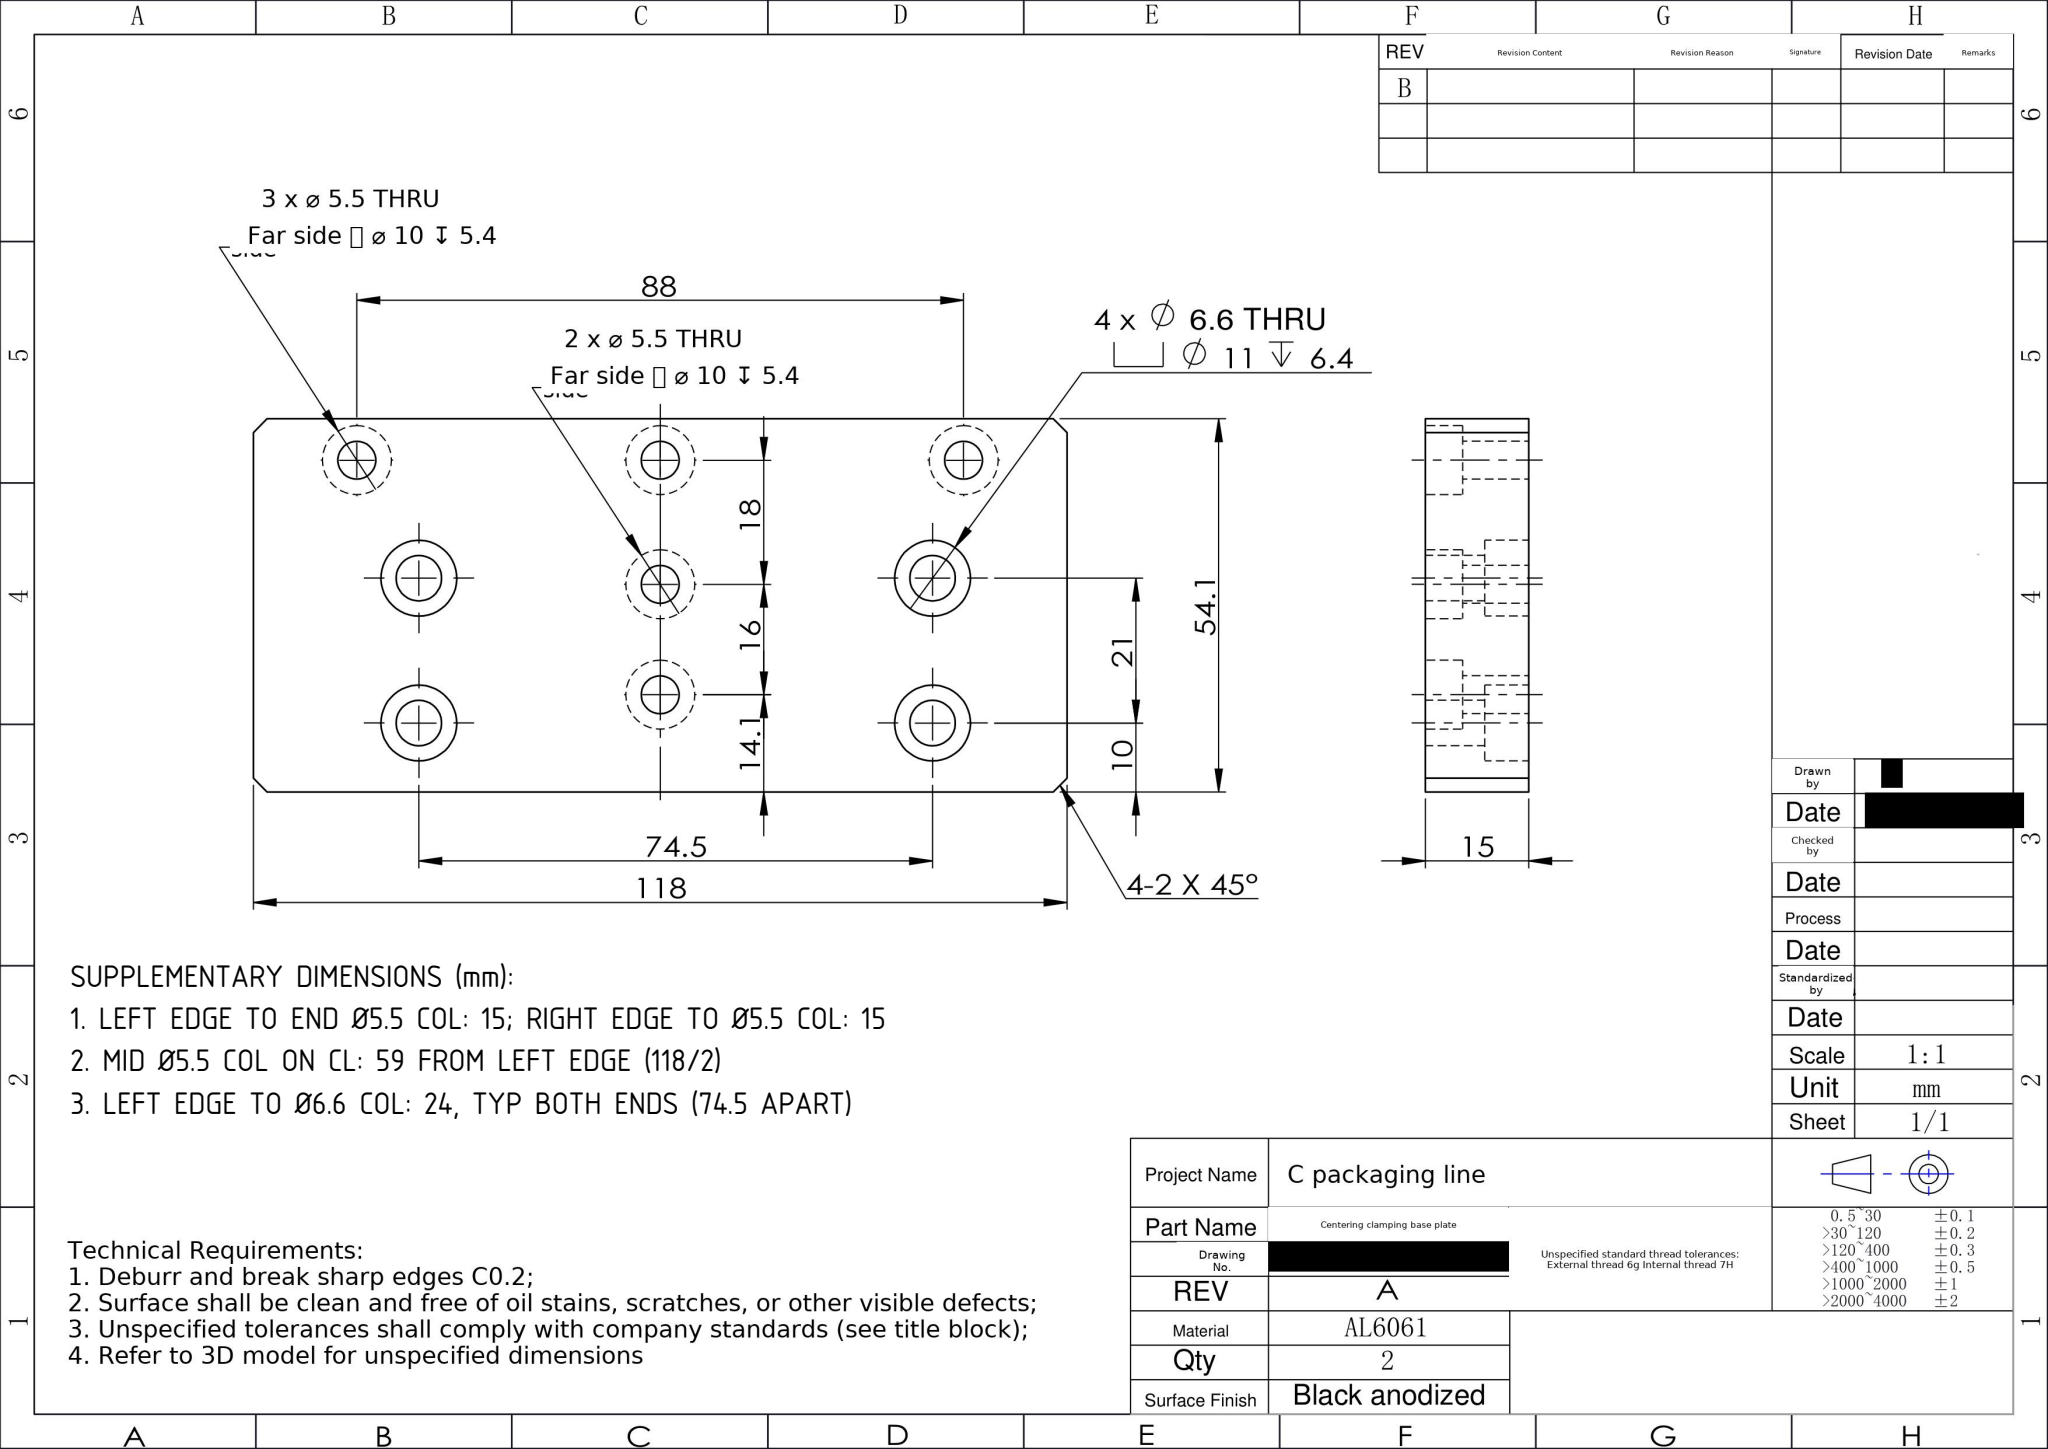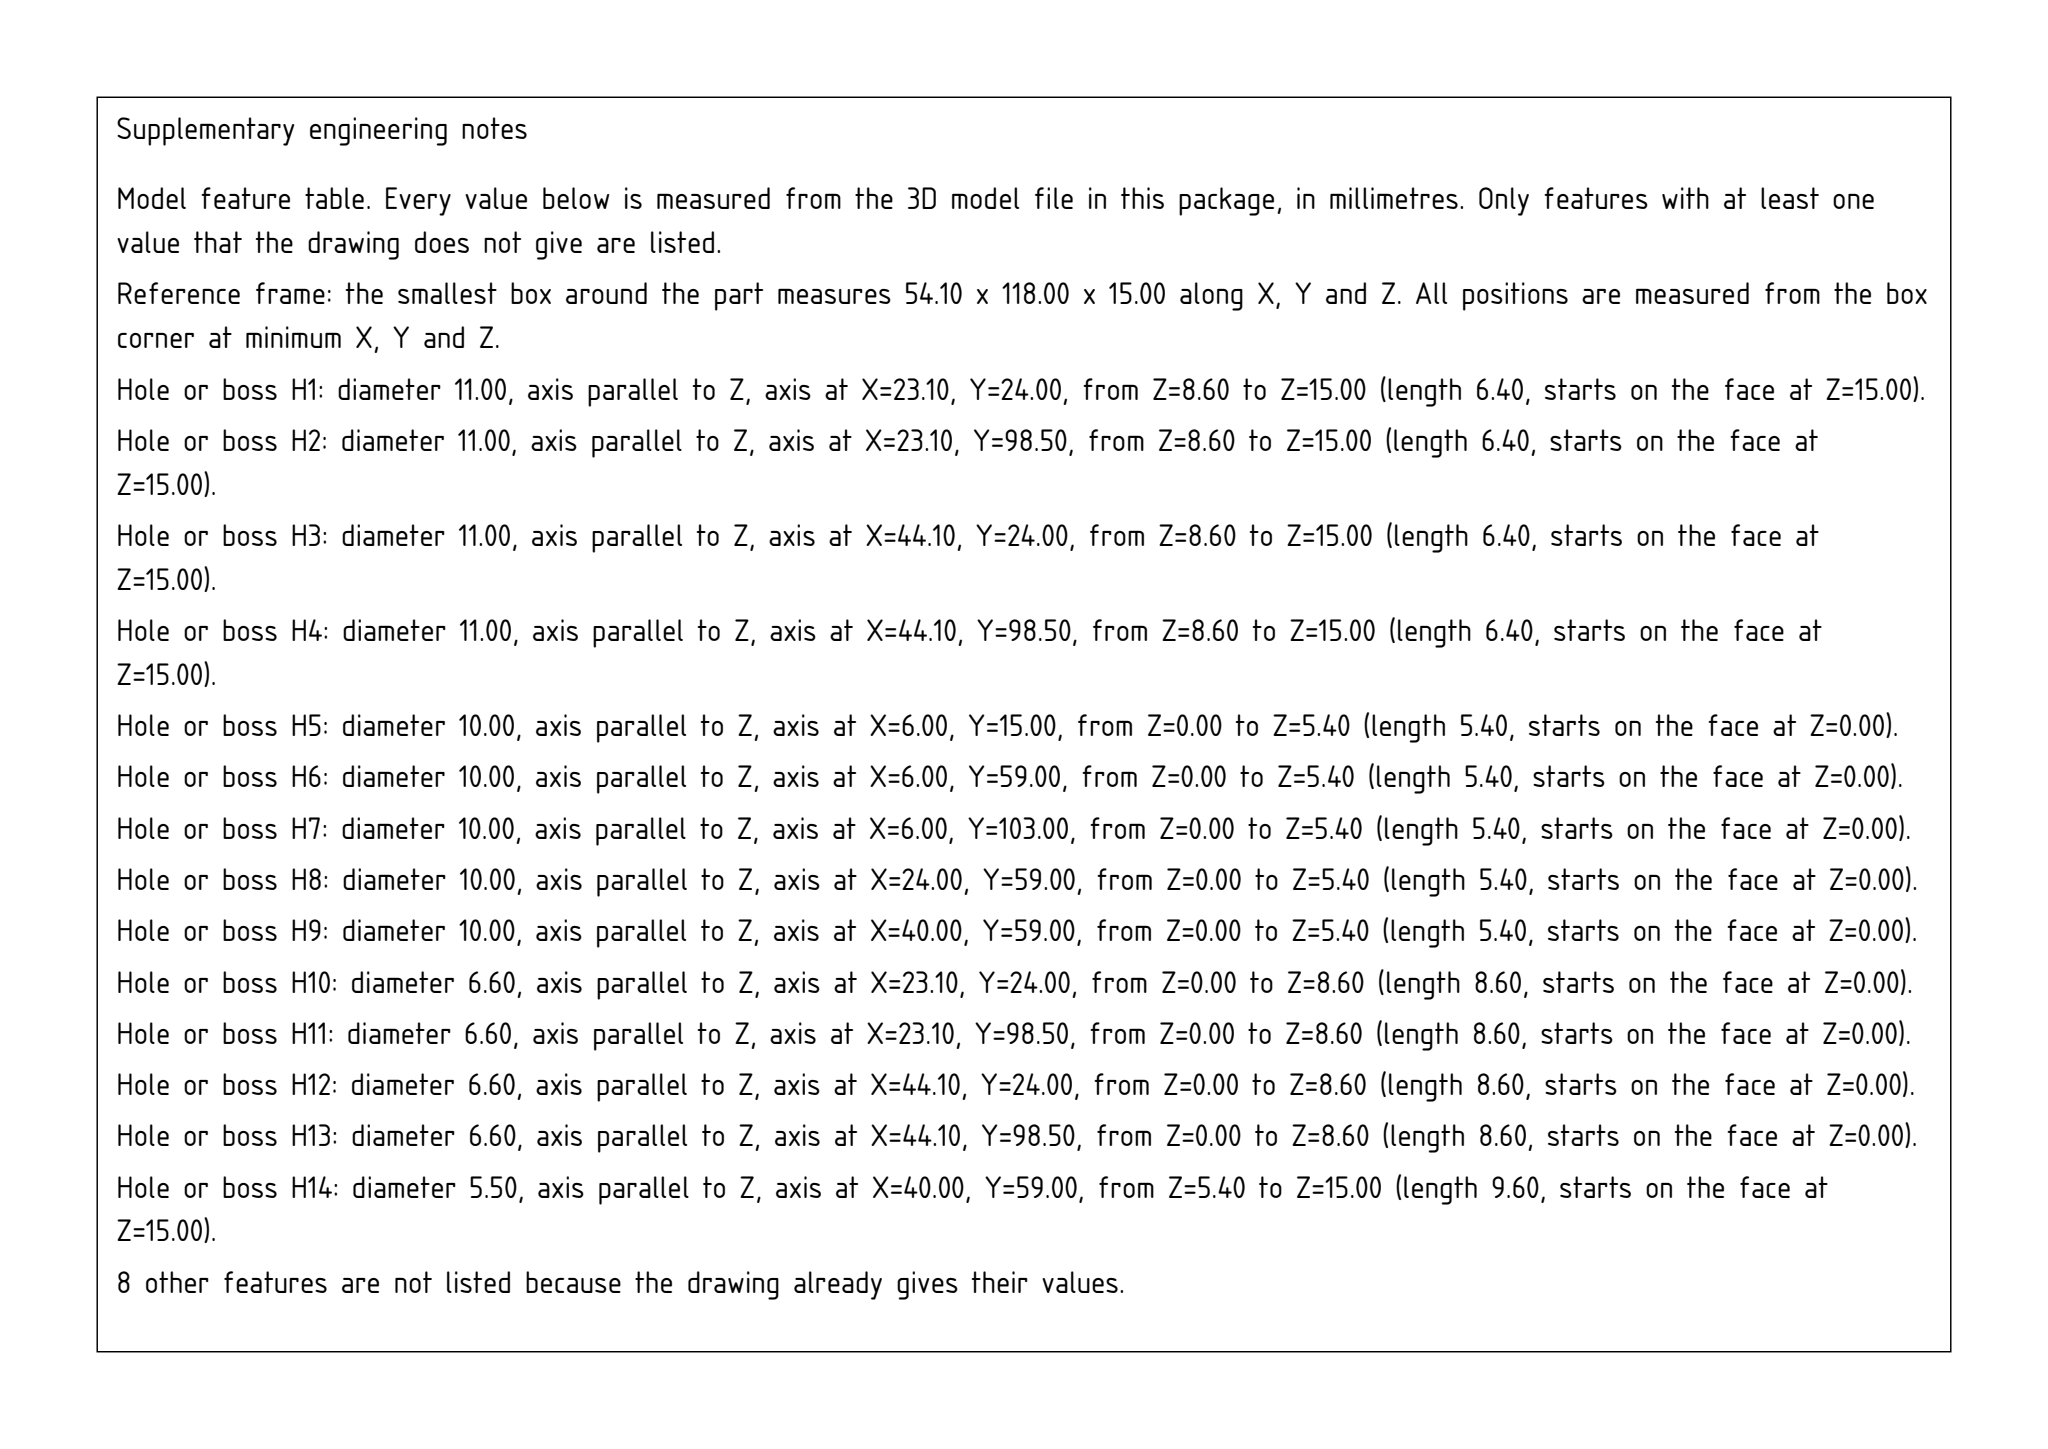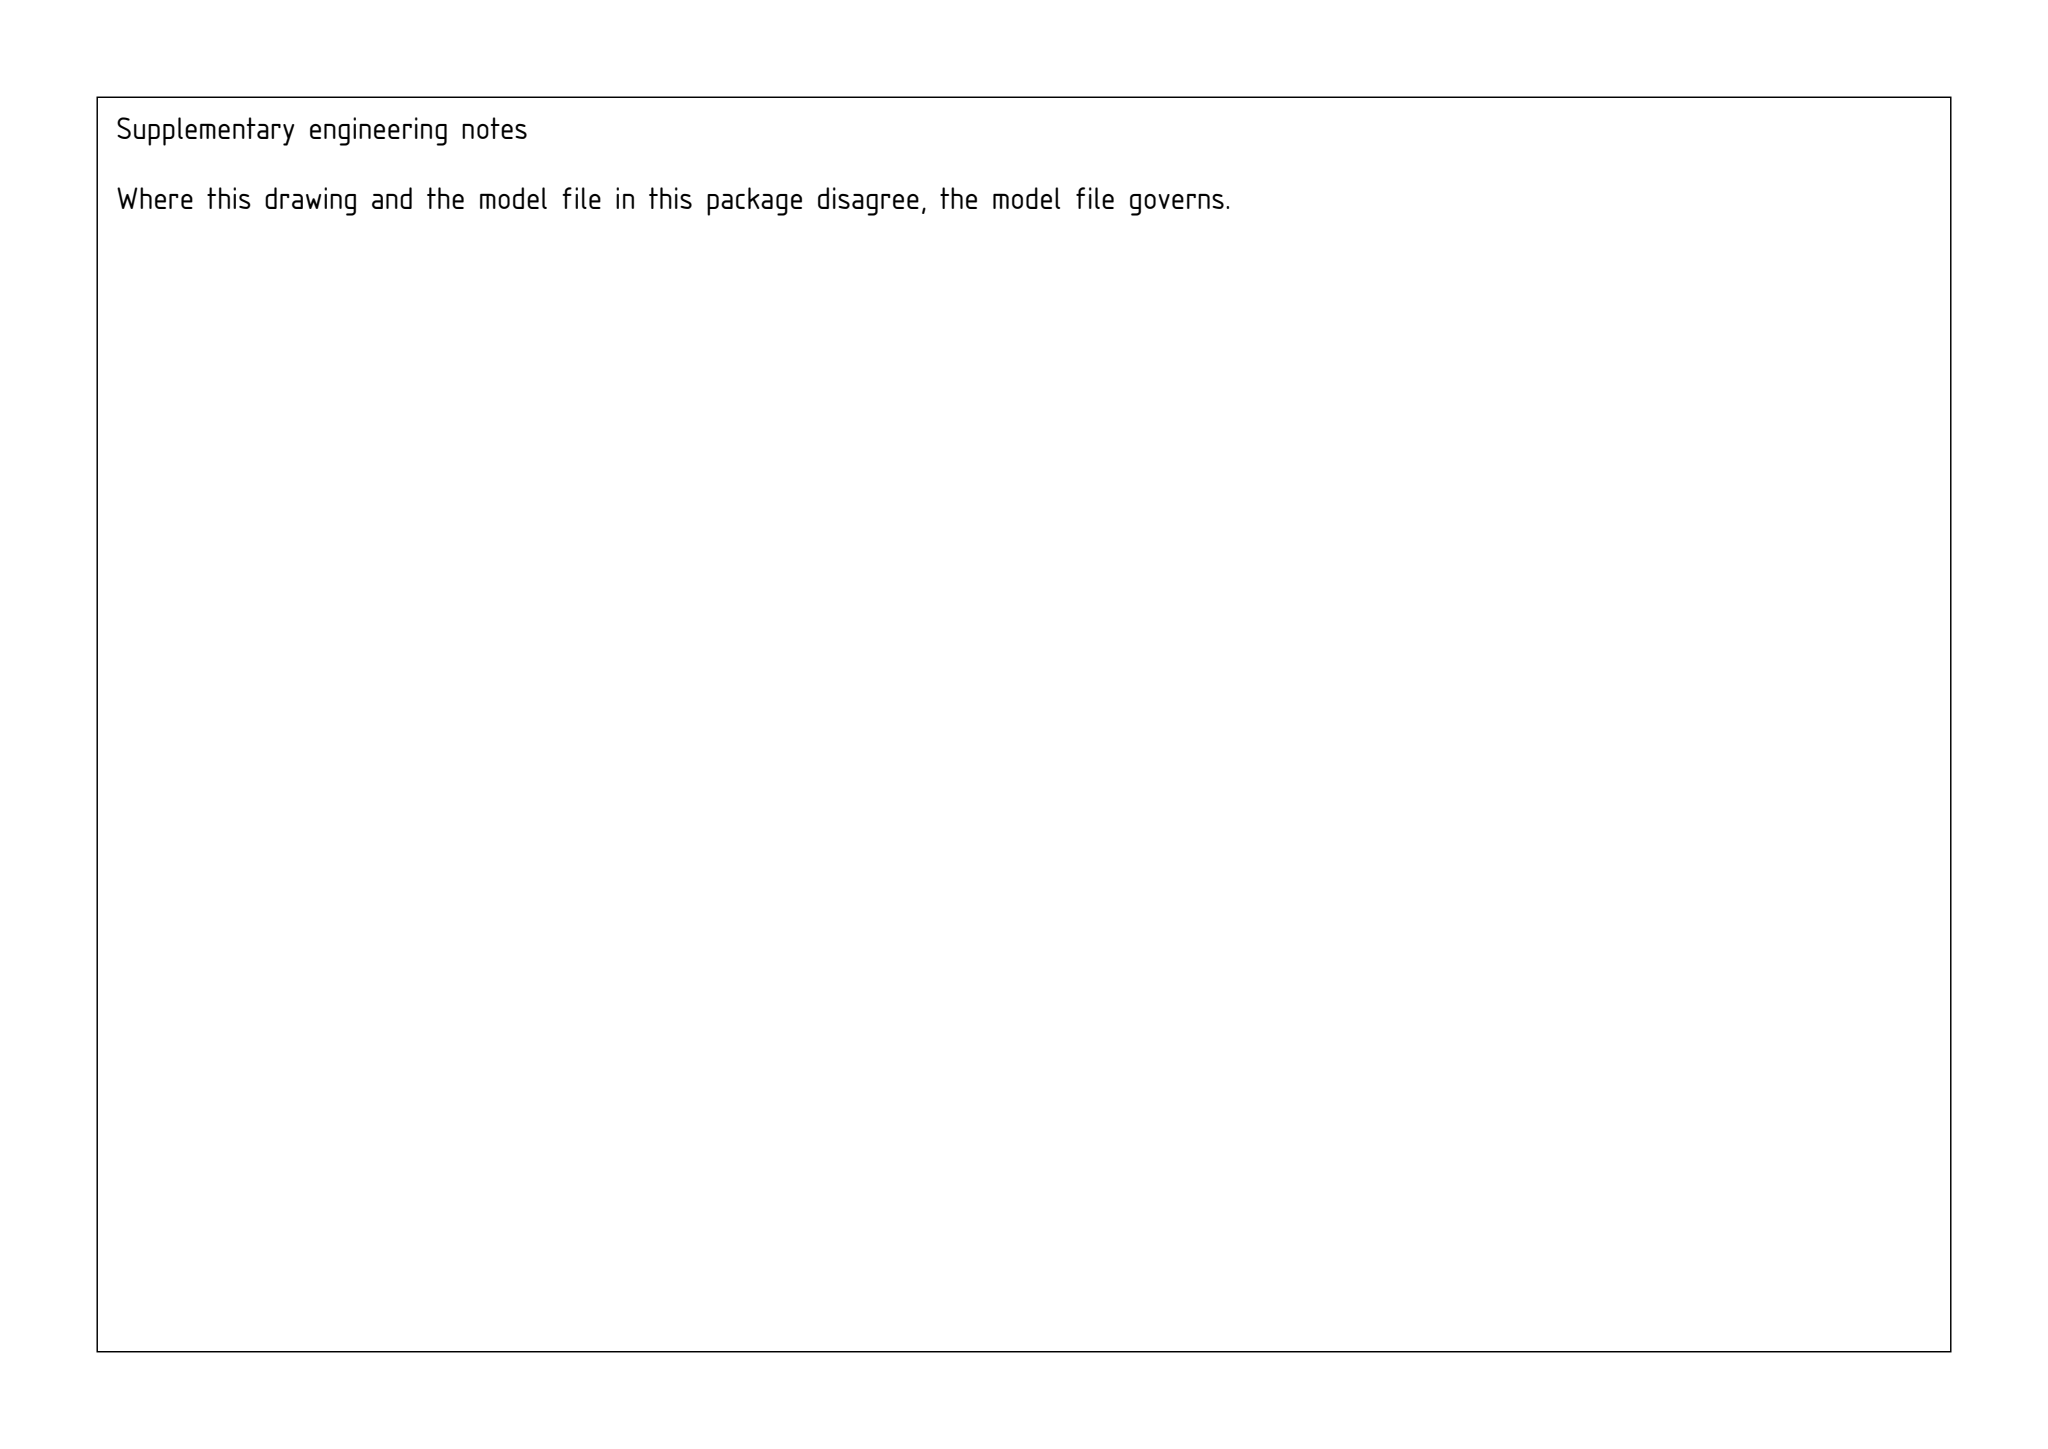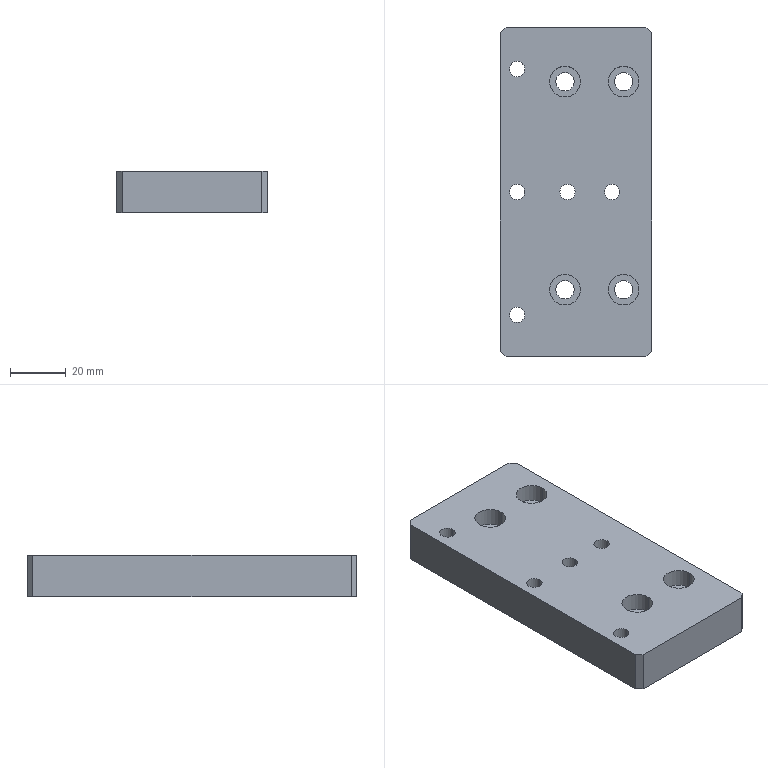Part | SolidWorks | mm | 1 solid | 55 faces | box 54.1 x 118 x 15 mm | volume 88766 mm3 | cylinder 36 | plane 19 | commonest cylinder face diameters 10 x10 5.5 x10 11 x8 6.6 x8
build123d program:
from build123d import *

# Parameters (mm, degrees)
SKETCH1_W                                       = 54.1
SKETCH1_H                                       = 118
BOSS_EXTRUDE1_DEPTH                             = 7.5
M6_HEX_SOCKET_HEAD_CAP_SCREW_CBORE1_D           = 6.6
M6_HEX_SOCKET_HEAD_CAP_SCREW_CBORE1_CBORE_D     = 11
M6_HEX_SOCKET_HEAD_CAP_SCREW_CBORE1_CBORE_DEPTH = 6.4
CHAMFER1_SIZE                                   = 2
M5_HEX_SOCKET_HEAD_CAP_SCREW_CBORE1_D           = 5.5
M5_HEX_SOCKET_HEAD_CAP_SCREW_CBORE1_CBORE_D     = 10
M5_HEX_SOCKET_HEAD_CAP_SCREW_CBORE1_CBORE_DEPTH = 5.4
M5_HEX_SOCKET_HEAD_CAP_SCREW_CBORE2_D           = 5.5
M5_HEX_SOCKET_HEAD_CAP_SCREW_CBORE2_CBORE_D     = 10
M5_HEX_SOCKET_HEAD_CAP_SCREW_CBORE2_CBORE_DEPTH = 5.4


with BuildPart() as part:
    # Sketch1 → Boss-Extrude1 (new, symmetric)
    with BuildSketch(Plane.XY):
        Rectangle(SKETCH1_W, SKETCH1_H)
    extrude(amount=BOSS_EXTRUDE1_DEPTH, both=True)

    # M6 Hex Socket Head Cap Screw CBORE1 (through all)
    with Locations(Plane.XY.offset(7.5)):
        with Locations((17.05, 39.5), (-3.95, -35), (-3.95, 39.5), (17.05, -35)):
            CounterBoreHole(M6_HEX_SOCKET_HEAD_CAP_SCREW_CBORE1_D / 2, M6_HEX_SOCKET_HEAD_CAP_SCREW_CBORE1_CBORE_D / 2, M6_HEX_SOCKET_HEAD_CAP_SCREW_CBORE1_CBORE_DEPTH)

    # Chamfer1
    chamfer1_edges = [part.edges().sort_by_distance(p)[0] for p in [
        (27.05, -59, 0),
        (-27.05, -59, 0),
        (-27.05, 59, 0),
        (27.05, 59, 0),
    ]]
    chamfer(chamfer1_edges, length=CHAMFER1_SIZE)

    # M5 Hex Socket Head Cap Screw CBORE1 (through all)
    with Locations(Plane(origin=(0, 0, -7.5), x_dir=(-1, 0, 0), z_dir=(0, 0, -1))):
        with Locations((3.05, 0), (-12.95, 0)):
            CounterBoreHole(M5_HEX_SOCKET_HEAD_CAP_SCREW_CBORE1_D / 2, M5_HEX_SOCKET_HEAD_CAP_SCREW_CBORE1_CBORE_D / 2, M5_HEX_SOCKET_HEAD_CAP_SCREW_CBORE1_CBORE_DEPTH)

    # M5 Hex Socket Head Cap Screw CBORE2 (through all)
    with Locations(Plane(origin=(0, 0, -7.5), x_dir=(-1, 0, 0), z_dir=(0, 0, -1))):
        with Locations((21.05, 44), (21.05, 0), (21.05, -44)):
            CounterBoreHole(M5_HEX_SOCKET_HEAD_CAP_SCREW_CBORE2_D / 2, M5_HEX_SOCKET_HEAD_CAP_SCREW_CBORE2_CBORE_D / 2, M5_HEX_SOCKET_HEAD_CAP_SCREW_CBORE2_CBORE_DEPTH)


solid = part.part